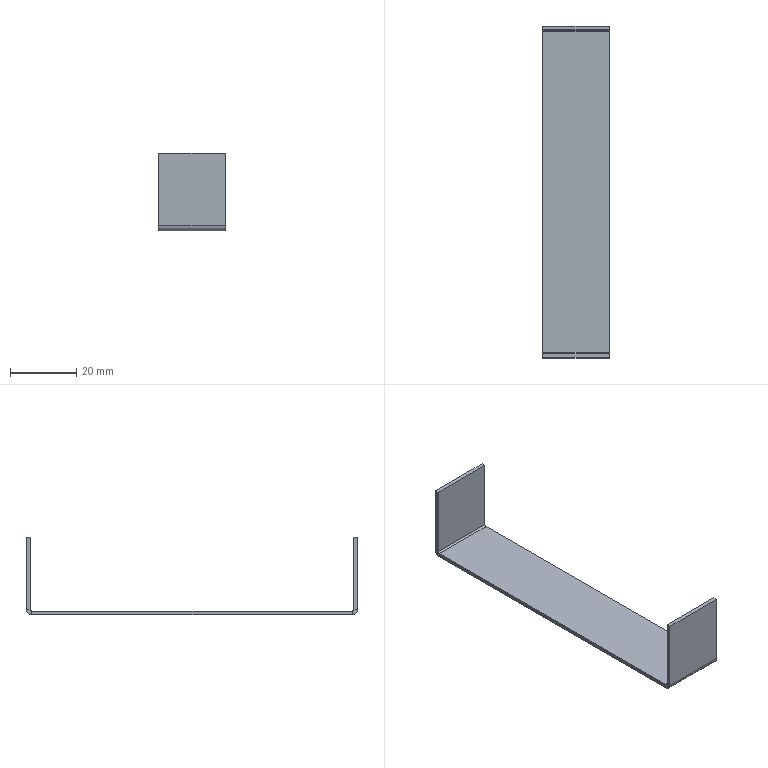Component | SolidWorks | AirFurnaceElectricalCabinet-DoorPanelAssembly-1_AirFurnaceElectricalCabinet-WiringBoard-2 | 1 solid | 22 faces | box 20 x 100 x 23.5 mm | volume 3448 mm3 | plane 18 | cylinder 4 | commonest cylinder face diameters 3.4 x2 1 x2
STEP:
#1=COLOUR_RGB('',0.7922,0.8196,0.9333);
#2=FILL_AREA_STYLE_COLOUR('',#1);
#3=FILL_AREA_STYLE('',(#2));
#4=SURFACE_STYLE_FILL_AREA(#3);
#5=SURFACE_SIDE_STYLE('',(#4));
#6=SURFACE_STYLE_USAGE(.BOTH.,#5);
#7=PRESENTATION_STYLE_ASSIGNMENT((#6));
#8=CARTESIAN_POINT('',(-18.504,43.728,9.055));
#9=VERTEX_POINT('',#8);
#10=CARTESIAN_POINT('',(-18.504,43.728,9.102));
#11=VERTEX_POINT('',#10);
#12=CARTESIAN_POINT('',(-18.504,43.728,9.055));
#13=DIRECTION('',(-0.,-0.,1.));
#14=VECTOR('',#13,39.37);
#15=LINE('',#12,#14);
#16=EDGE_CURVE('',#9,#11,#15,.T.);
#17=ORIENTED_EDGE('',*,*,#16,.F.);
#18=CARTESIAN_POINT('',(-18.504,43.661,9.122));
#19=VERTEX_POINT('',#18);
#20=CARTESIAN_POINT('',(-18.504,43.728,9.122));
#21=DIRECTION('',(1.,-0.,0.));
#22=DIRECTION('',(0.,1.,0.));
#23=AXIS2_PLACEMENT_3D('',#20,#21,#22);
#24=CIRCLE('',#23,0.06693);
#25=EDGE_CURVE('',#19,#9,#24,.T.);
#26=ORIENTED_EDGE('',*,*,#25,.F.);
#27=CARTESIAN_POINT('',(-18.504,43.709,9.122));
#28=VERTEX_POINT('',#27);
#29=CARTESIAN_POINT('',(-18.504,43.709,9.122));
#30=DIRECTION('',(-0.,-1.,-0.));
#31=VECTOR('',#30,39.37);
#32=LINE('',#29,#31);
#33=EDGE_CURVE('',#28,#19,#32,.T.);
#34=ORIENTED_EDGE('',*,*,#33,.F.);
#35=CARTESIAN_POINT('',(-18.504,43.728,9.122));
#36=DIRECTION('',(1.,-0.,0.));
#37=DIRECTION('',(0.,1.,0.));
#38=AXIS2_PLACEMENT_3D('',#35,#36,#37);
#39=CIRCLE('',#38,0.01969);
#40=EDGE_CURVE('',#28,#11,#39,.T.);
#41=ORIENTED_EDGE('',*,*,#40,.T.);
#42=EDGE_LOOP('',(#17,#26,#34,#41));
#43=FACE_OUTER_BOUND('',#42,.T.);
#44=CARTESIAN_POINT('',(-18.504,43.728,9.055));
#45=DIRECTION('',(-1.,0.,-0.));
#46=DIRECTION('',(0.,1.,0.));
#47=AXIS2_PLACEMENT_3D('',#44,#45,#46);
#48=PLANE('',#47);
#49=ADVANCED_FACE('',(#43),#48,.T.);
#50=CARTESIAN_POINT('',(-18.504,47.531,9.055));
#51=VERTEX_POINT('',#50);
#52=CARTESIAN_POINT('',(-18.504,43.661,9.055));
#53=DIRECTION('',(0.,1.,0.));
#54=VECTOR('',#53,39.37);
#55=LINE('',#52,#54);
#56=EDGE_CURVE('',#9,#51,#55,.T.);
#57=ORIENTED_EDGE('',*,*,#56,.F.);
#58=ORIENTED_EDGE('',*,*,#16,.T.);
#59=CARTESIAN_POINT('',(-18.504,47.531,9.102));
#60=VERTEX_POINT('',#59);
#61=CARTESIAN_POINT('',(-18.504,43.661,9.102));
#62=DIRECTION('',(0.,1.,0.));
#63=VECTOR('',#62,39.37);
#64=LINE('',#61,#63);
#65=EDGE_CURVE('',#11,#60,#64,.T.);
#66=ORIENTED_EDGE('',*,*,#65,.T.);
#67=CARTESIAN_POINT('',(-18.504,47.531,9.102));
#68=DIRECTION('',(0.,0.,-1.));
#69=VECTOR('',#68,39.37);
#70=LINE('',#67,#69);
#71=EDGE_CURVE('',#60,#51,#70,.T.);
#72=ORIENTED_EDGE('',*,*,#71,.T.);
#73=EDGE_LOOP('',(#57,#58,#66,#72));
#74=FACE_OUTER_BOUND('',#73,.T.);
#75=CARTESIAN_POINT('',(-18.504,43.709,9.122));
#76=DIRECTION('',(-1.,0.,-0.));
#77=DIRECTION('',(0.,1.,0.));
#78=AXIS2_PLACEMENT_3D('',#75,#76,#77);
#79=PLANE('',#78);
#80=ADVANCED_FACE('',(#74),#79,.T.);
#81=CARTESIAN_POINT('',(-17.717,43.661,9.122));
#82=VERTEX_POINT('',#81);
#83=CARTESIAN_POINT('',(-17.717,43.709,9.122));
#84=VERTEX_POINT('',#83);
#85=CARTESIAN_POINT('',(-17.717,43.661,9.122));
#86=DIRECTION('',(0.,1.,0.));
#87=VECTOR('',#86,39.37);
#88=LINE('',#85,#87);
#89=EDGE_CURVE('',#82,#84,#88,.T.);
#90=ORIENTED_EDGE('',*,*,#89,.F.);
#91=CARTESIAN_POINT('',(-17.717,43.728,9.055));
#92=VERTEX_POINT('',#91);
#93=CARTESIAN_POINT('',(-17.717,43.728,9.122));
#94=DIRECTION('',(1.,-0.,0.));
#95=DIRECTION('',(0.,1.,0.));
#96=AXIS2_PLACEMENT_3D('',#93,#94,#95);
#97=CIRCLE('',#96,0.06693);
#98=EDGE_CURVE('',#82,#92,#97,.T.);
#99=ORIENTED_EDGE('',*,*,#98,.T.);
#100=CARTESIAN_POINT('',(-17.717,43.728,9.102));
#101=VERTEX_POINT('',#100);
#102=CARTESIAN_POINT('',(-17.717,43.728,9.102));
#103=DIRECTION('',(0.,0.,-1.));
#104=VECTOR('',#103,39.37);
#105=LINE('',#102,#104);
#106=EDGE_CURVE('',#101,#92,#105,.T.);
#107=ORIENTED_EDGE('',*,*,#106,.F.);
#108=CARTESIAN_POINT('',(-17.717,43.728,9.122));
#109=DIRECTION('',(1.,-0.,0.));
#110=DIRECTION('',(0.,1.,0.));
#111=AXIS2_PLACEMENT_3D('',#108,#109,#110);
#112=CIRCLE('',#111,0.01969);
#113=EDGE_CURVE('',#84,#101,#112,.T.);
#114=ORIENTED_EDGE('',*,*,#113,.F.);
#115=EDGE_LOOP('',(#90,#99,#107,#114));
#116=FACE_OUTER_BOUND('',#115,.T.);
#117=CARTESIAN_POINT('',(-17.717,43.661,9.122));
#118=DIRECTION('',(1.,-0.,0.));
#119=DIRECTION('',(-0.,-1.,-0.));
#120=AXIS2_PLACEMENT_3D('',#117,#118,#119);
#121=PLANE('',#120);
#122=ADVANCED_FACE('',(#116),#121,.T.);
#123=CARTESIAN_POINT('',(-17.717,43.661,9.98));
#124=VERTEX_POINT('',#123);
#125=CARTESIAN_POINT('',(-17.717,43.661,9.98));
#126=DIRECTION('',(0.,0.,-1.));
#127=VECTOR('',#126,39.37);
#128=LINE('',#125,#127);
#129=EDGE_CURVE('',#124,#82,#128,.T.);
#130=ORIENTED_EDGE('',*,*,#129,.T.);
#131=ORIENTED_EDGE('',*,*,#89,.T.);
#132=CARTESIAN_POINT('',(-17.717,43.709,9.98));
#133=VERTEX_POINT('',#132);
#134=CARTESIAN_POINT('',(-17.717,43.709,9.98));
#135=DIRECTION('',(0.,0.,-1.));
#136=VECTOR('',#135,39.37);
#137=LINE('',#134,#136);
#138=EDGE_CURVE('',#133,#84,#137,.T.);
#139=ORIENTED_EDGE('',*,*,#138,.F.);
#140=CARTESIAN_POINT('',(-17.717,43.709,9.98));
#141=DIRECTION('',(-0.,-1.,-0.));
#142=VECTOR('',#141,39.37);
#143=LINE('',#140,#142);
#144=EDGE_CURVE('',#133,#124,#143,.T.);
#145=ORIENTED_EDGE('',*,*,#144,.T.);
#146=EDGE_LOOP('',(#130,#131,#139,#145));
#147=FACE_OUTER_BOUND('',#146,.T.);
#148=CARTESIAN_POINT('',(-17.717,43.728,9.102));
#149=DIRECTION('',(1.,-0.,0.));
#150=DIRECTION('',(-0.,-1.,-0.));
#151=AXIS2_PLACEMENT_3D('',#148,#149,#150);
#152=PLANE('',#151);
#153=ADVANCED_FACE('',(#147),#152,.T.);
#154=CARTESIAN_POINT('',(-18.504,47.598,9.122));
#155=VERTEX_POINT('',#154);
#156=CARTESIAN_POINT('',(-18.504,47.551,9.122));
#157=VERTEX_POINT('',#156);
#158=CARTESIAN_POINT('',(-18.504,47.598,9.122));
#159=DIRECTION('',(-0.,-1.,-0.));
#160=VECTOR('',#159,39.37);
#161=LINE('',#158,#160);
#162=EDGE_CURVE('',#155,#157,#161,.T.);
#163=ORIENTED_EDGE('',*,*,#162,.F.);
#164=CARTESIAN_POINT('',(-18.504,47.531,9.122));
#165=DIRECTION('',(1.,-0.,0.));
#166=DIRECTION('',(0.,1.,0.));
#167=AXIS2_PLACEMENT_3D('',#164,#165,#166);
#168=CIRCLE('',#167,0.06693);
#169=EDGE_CURVE('',#51,#155,#168,.T.);
#170=ORIENTED_EDGE('',*,*,#169,.F.);
#171=ORIENTED_EDGE('',*,*,#71,.F.);
#172=CARTESIAN_POINT('',(-18.504,47.531,9.122));
#173=DIRECTION('',(1.,-0.,0.));
#174=DIRECTION('',(0.,1.,0.));
#175=AXIS2_PLACEMENT_3D('',#172,#173,#174);
#176=CIRCLE('',#175,0.01969);
#177=EDGE_CURVE('',#60,#157,#176,.T.);
#178=ORIENTED_EDGE('',*,*,#177,.T.);
#179=EDGE_LOOP('',(#163,#170,#171,#178));
#180=FACE_OUTER_BOUND('',#179,.T.);
#181=CARTESIAN_POINT('',(-18.504,47.598,9.122));
#182=DIRECTION('',(-1.,0.,-0.));
#183=DIRECTION('',(0.,1.,0.));
#184=AXIS2_PLACEMENT_3D('',#181,#182,#183);
#185=PLANE('',#184);
#186=ADVANCED_FACE('',(#180),#185,.T.);
#187=CARTESIAN_POINT('',(-18.504,47.598,9.98));
#188=VERTEX_POINT('',#187);
#189=CARTESIAN_POINT('',(-18.504,47.598,9.055));
#190=DIRECTION('',(-0.,-0.,1.));
#191=VECTOR('',#190,39.37);
#192=LINE('',#189,#191);
#193=EDGE_CURVE('',#155,#188,#192,.T.);
#194=ORIENTED_EDGE('',*,*,#193,.F.);
#195=ORIENTED_EDGE('',*,*,#162,.T.);
#196=CARTESIAN_POINT('',(-18.504,47.551,9.98));
#197=VERTEX_POINT('',#196);
#198=CARTESIAN_POINT('',(-18.504,47.551,9.055));
#199=DIRECTION('',(-0.,-0.,1.));
#200=VECTOR('',#199,39.37);
#201=LINE('',#198,#200);
#202=EDGE_CURVE('',#157,#197,#201,.T.);
#203=ORIENTED_EDGE('',*,*,#202,.T.);
#204=CARTESIAN_POINT('',(-18.504,47.598,9.98));
#205=DIRECTION('',(-0.,-1.,-0.));
#206=VECTOR('',#205,39.37);
#207=LINE('',#204,#206);
#208=EDGE_CURVE('',#188,#197,#207,.T.);
#209=ORIENTED_EDGE('',*,*,#208,.F.);
#210=EDGE_LOOP('',(#194,#195,#203,#209));
#211=FACE_OUTER_BOUND('',#210,.T.);
#212=CARTESIAN_POINT('',(-18.504,47.531,9.102));
#213=DIRECTION('',(-1.,0.,-0.));
#214=DIRECTION('',(0.,1.,0.));
#215=AXIS2_PLACEMENT_3D('',#212,#213,#214);
#216=PLANE('',#215);
#217=ADVANCED_FACE('',(#211),#216,.T.);
#218=CARTESIAN_POINT('',(-17.717,47.531,9.055));
#219=VERTEX_POINT('',#218);
#220=CARTESIAN_POINT('',(-17.717,47.531,9.102));
#221=VERTEX_POINT('',#220);
#222=CARTESIAN_POINT('',(-17.717,47.531,9.055));
#223=DIRECTION('',(-0.,-0.,1.));
#224=VECTOR('',#223,39.37);
#225=LINE('',#222,#224);
#226=EDGE_CURVE('',#219,#221,#225,.T.);
#227=ORIENTED_EDGE('',*,*,#226,.F.);
#228=CARTESIAN_POINT('',(-17.717,47.598,9.122));
#229=VERTEX_POINT('',#228);
#230=CARTESIAN_POINT('',(-17.717,47.531,9.122));
#231=DIRECTION('',(1.,-0.,0.));
#232=DIRECTION('',(0.,1.,0.));
#233=AXIS2_PLACEMENT_3D('',#230,#231,#232);
#234=CIRCLE('',#233,0.06693);
#235=EDGE_CURVE('',#219,#229,#234,.T.);
#236=ORIENTED_EDGE('',*,*,#235,.T.);
#237=CARTESIAN_POINT('',(-17.717,47.551,9.122));
#238=VERTEX_POINT('',#237);
#239=CARTESIAN_POINT('',(-17.717,47.551,9.122));
#240=DIRECTION('',(0.,1.,0.));
#241=VECTOR('',#240,39.37);
#242=LINE('',#239,#241);
#243=EDGE_CURVE('',#238,#229,#242,.T.);
#244=ORIENTED_EDGE('',*,*,#243,.F.);
#245=CARTESIAN_POINT('',(-17.717,47.531,9.122));
#246=DIRECTION('',(1.,-0.,0.));
#247=DIRECTION('',(0.,1.,0.));
#248=AXIS2_PLACEMENT_3D('',#245,#246,#247);
#249=CIRCLE('',#248,0.01969);
#250=EDGE_CURVE('',#221,#238,#249,.T.);
#251=ORIENTED_EDGE('',*,*,#250,.F.);
#252=EDGE_LOOP('',(#227,#236,#244,#251));
#253=FACE_OUTER_BOUND('',#252,.T.);
#254=CARTESIAN_POINT('',(-17.717,47.531,9.055));
#255=DIRECTION('',(1.,-0.,0.));
#256=DIRECTION('',(-0.,-1.,-0.));
#257=AXIS2_PLACEMENT_3D('',#254,#255,#256);
#258=PLANE('',#257);
#259=ADVANCED_FACE('',(#253),#258,.T.);
#260=CARTESIAN_POINT('',(-17.717,43.661,9.055));
#261=DIRECTION('',(0.,1.,0.));
#262=VECTOR('',#261,39.37);
#263=LINE('',#260,#262);
#264=EDGE_CURVE('',#92,#219,#263,.T.);
#265=ORIENTED_EDGE('',*,*,#264,.T.);
#266=ORIENTED_EDGE('',*,*,#226,.T.);
#267=CARTESIAN_POINT('',(-17.717,43.661,9.102));
#268=DIRECTION('',(0.,1.,0.));
#269=VECTOR('',#268,39.37);
#270=LINE('',#267,#269);
#271=EDGE_CURVE('',#101,#221,#270,.T.);
#272=ORIENTED_EDGE('',*,*,#271,.F.);
#273=ORIENTED_EDGE('',*,*,#106,.T.);
#274=EDGE_LOOP('',(#265,#266,#272,#273));
#275=FACE_OUTER_BOUND('',#274,.T.);
#276=CARTESIAN_POINT('',(-17.717,47.551,9.122));
#277=DIRECTION('',(1.,-0.,0.));
#278=DIRECTION('',(-0.,-1.,-0.));
#279=AXIS2_PLACEMENT_3D('',#276,#277,#278);
#280=PLANE('',#279);
#281=ADVANCED_FACE('',(#275),#280,.T.);
#282=CARTESIAN_POINT('',(-17.717,47.551,9.98));
#283=VERTEX_POINT('',#282);
#284=CARTESIAN_POINT('',(-17.717,47.551,9.055));
#285=DIRECTION('',(-0.,-0.,1.));
#286=VECTOR('',#285,39.37);
#287=LINE('',#284,#286);
#288=EDGE_CURVE('',#238,#283,#287,.T.);
#289=ORIENTED_EDGE('',*,*,#288,.T.);
#290=CARTESIAN_POINT('',(-18.504,47.551,9.98));
#291=DIRECTION('',(1.,-0.,0.));
#292=VECTOR('',#291,39.37);
#293=LINE('',#290,#292);
#294=EDGE_CURVE('',#197,#283,#293,.T.);
#295=ORIENTED_EDGE('',*,*,#294,.F.);
#296=ORIENTED_EDGE('',*,*,#202,.F.);
#297=CARTESIAN_POINT('',(-18.504,47.551,9.122));
#298=DIRECTION('',(1.,-0.,0.));
#299=VECTOR('',#298,39.37);
#300=LINE('',#297,#299);
#301=EDGE_CURVE('',#157,#238,#300,.T.);
#302=ORIENTED_EDGE('',*,*,#301,.T.);
#303=EDGE_LOOP('',(#289,#295,#296,#302));
#304=FACE_OUTER_BOUND('',#303,.T.);
#305=CARTESIAN_POINT('',(-18.504,47.551,9.055));
#306=DIRECTION('',(0.,1.,0.));
#307=DIRECTION('',(0.,0.,-1.));
#308=AXIS2_PLACEMENT_3D('',#305,#306,#307);
#309=PLANE('',#308);
#310=ADVANCED_FACE('',(#304),#309,.F.);
#311=CARTESIAN_POINT('',(-17.717,47.598,9.98));
#312=VERTEX_POINT('',#311);
#313=CARTESIAN_POINT('',(-17.717,47.598,9.98));
#314=DIRECTION('',(-0.,-1.,-0.));
#315=VECTOR('',#314,39.37);
#316=LINE('',#313,#315);
#317=EDGE_CURVE('',#312,#283,#316,.T.);
#318=ORIENTED_EDGE('',*,*,#317,.F.);
#319=CARTESIAN_POINT('',(-18.504,47.598,9.98));
#320=DIRECTION('',(1.,-0.,0.));
#321=VECTOR('',#320,39.37);
#322=LINE('',#319,#321);
#323=EDGE_CURVE('',#188,#312,#322,.T.);
#324=ORIENTED_EDGE('',*,*,#323,.F.);
#325=ORIENTED_EDGE('',*,*,#208,.T.);
#326=ORIENTED_EDGE('',*,*,#294,.T.);
#327=EDGE_LOOP('',(#318,#324,#325,#326));
#328=FACE_OUTER_BOUND('',#327,.T.);
#329=CARTESIAN_POINT('',(-18.504,47.598,9.98));
#330=DIRECTION('',(-0.,-0.,1.));
#331=DIRECTION('',(0.,1.,0.));
#332=AXIS2_PLACEMENT_3D('',#329,#330,#331);
#333=PLANE('',#332);
#334=ADVANCED_FACE('',(#328),#333,.T.);
#335=CARTESIAN_POINT('',(-17.717,47.598,9.055));
#336=DIRECTION('',(-0.,-0.,1.));
#337=VECTOR('',#336,39.37);
#338=LINE('',#335,#337);
#339=EDGE_CURVE('',#229,#312,#338,.T.);
#340=ORIENTED_EDGE('',*,*,#339,.F.);
#341=CARTESIAN_POINT('',(-18.504,47.598,9.122));
#342=DIRECTION('',(1.,-0.,0.));
#343=VECTOR('',#342,39.37);
#344=LINE('',#341,#343);
#345=EDGE_CURVE('',#155,#229,#344,.T.);
#346=ORIENTED_EDGE('',*,*,#345,.F.);
#347=ORIENTED_EDGE('',*,*,#193,.T.);
#348=ORIENTED_EDGE('',*,*,#323,.T.);
#349=EDGE_LOOP('',(#340,#346,#347,#348));
#350=FACE_OUTER_BOUND('',#349,.T.);
#351=CARTESIAN_POINT('',(-18.504,47.598,9.055));
#352=DIRECTION('',(0.,1.,0.));
#353=DIRECTION('',(0.,0.,-1.));
#354=AXIS2_PLACEMENT_3D('',#351,#352,#353);
#355=PLANE('',#354);
#356=ADVANCED_FACE('',(#350),#355,.T.);
#357=ORIENTED_EDGE('',*,*,#235,.F.);
#358=CARTESIAN_POINT('',(-18.504,47.531,9.055));
#359=DIRECTION('',(1.,-0.,0.));
#360=VECTOR('',#359,39.37);
#361=LINE('',#358,#360);
#362=EDGE_CURVE('',#51,#219,#361,.T.);
#363=ORIENTED_EDGE('',*,*,#362,.F.);
#364=ORIENTED_EDGE('',*,*,#169,.T.);
#365=ORIENTED_EDGE('',*,*,#345,.T.);
#366=EDGE_LOOP('',(#357,#363,#364,#365));
#367=FACE_OUTER_BOUND('',#366,.T.);
#368=CARTESIAN_POINT('',(-18.504,47.531,9.122));
#369=DIRECTION('',(1.,-0.,0.));
#370=DIRECTION('',(0.,-1.,0.));
#371=AXIS2_PLACEMENT_3D('',#368,#369,#370);
#372=CYLINDRICAL_SURFACE('',#371,0.06693);
#373=ADVANCED_FACE('',(#367),#372,.T.);
#374=ORIENTED_EDGE('',*,*,#264,.F.);
#375=CARTESIAN_POINT('',(-18.504,43.728,9.055));
#376=DIRECTION('',(1.,-0.,0.));
#377=VECTOR('',#376,39.37);
#378=LINE('',#375,#377);
#379=EDGE_CURVE('',#9,#92,#378,.T.);
#380=ORIENTED_EDGE('',*,*,#379,.F.);
#381=ORIENTED_EDGE('',*,*,#56,.T.);
#382=ORIENTED_EDGE('',*,*,#362,.T.);
#383=EDGE_LOOP('',(#374,#380,#381,#382));
#384=FACE_OUTER_BOUND('',#383,.T.);
#385=CARTESIAN_POINT('',(-18.504,43.661,9.055));
#386=DIRECTION('',(0.,0.,-1.));
#387=DIRECTION('',(-0.,-1.,-0.));
#388=AXIS2_PLACEMENT_3D('',#385,#386,#387);
#389=PLANE('',#388);
#390=ADVANCED_FACE('',(#384),#389,.T.);
#391=ORIENTED_EDGE('',*,*,#98,.F.);
#392=CARTESIAN_POINT('',(-18.504,43.661,9.122));
#393=DIRECTION('',(1.,-0.,0.));
#394=VECTOR('',#393,39.37);
#395=LINE('',#392,#394);
#396=EDGE_CURVE('',#19,#82,#395,.T.);
#397=ORIENTED_EDGE('',*,*,#396,.F.);
#398=ORIENTED_EDGE('',*,*,#25,.T.);
#399=ORIENTED_EDGE('',*,*,#379,.T.);
#400=EDGE_LOOP('',(#391,#397,#398,#399));
#401=FACE_OUTER_BOUND('',#400,.T.);
#402=CARTESIAN_POINT('',(-18.504,43.728,9.122));
#403=DIRECTION('',(1.,-0.,0.));
#404=DIRECTION('',(0.,-1.,0.));
#405=AXIS2_PLACEMENT_3D('',#402,#403,#404);
#406=CYLINDRICAL_SURFACE('',#405,0.06693);
#407=ADVANCED_FACE('',(#401),#406,.T.);
#408=ORIENTED_EDGE('',*,*,#129,.F.);
#409=CARTESIAN_POINT('',(-18.504,43.661,9.98));
#410=VERTEX_POINT('',#409);
#411=CARTESIAN_POINT('',(-18.504,43.661,9.98));
#412=DIRECTION('',(1.,-0.,0.));
#413=VECTOR('',#412,39.37);
#414=LINE('',#411,#413);
#415=EDGE_CURVE('',#410,#124,#414,.T.);
#416=ORIENTED_EDGE('',*,*,#415,.F.);
#417=CARTESIAN_POINT('',(-18.504,43.661,9.98));
#418=DIRECTION('',(0.,0.,-1.));
#419=VECTOR('',#418,39.37);
#420=LINE('',#417,#419);
#421=EDGE_CURVE('',#410,#19,#420,.T.);
#422=ORIENTED_EDGE('',*,*,#421,.T.);
#423=ORIENTED_EDGE('',*,*,#396,.T.);
#424=EDGE_LOOP('',(#408,#416,#422,#423));
#425=FACE_OUTER_BOUND('',#424,.T.);
#426=CARTESIAN_POINT('',(-18.504,43.661,9.98));
#427=DIRECTION('',(0.,-1.,-0.));
#428=DIRECTION('',(-1.,0.,-0.));
#429=AXIS2_PLACEMENT_3D('',#426,#427,#428);
#430=PLANE('',#429);
#431=ADVANCED_FACE('',(#425),#430,.T.);
#432=ORIENTED_EDGE('',*,*,#144,.F.);
#433=CARTESIAN_POINT('',(-18.504,43.709,9.98));
#434=VERTEX_POINT('',#433);
#435=CARTESIAN_POINT('',(-18.504,43.709,9.98));
#436=DIRECTION('',(1.,-0.,0.));
#437=VECTOR('',#436,39.37);
#438=LINE('',#435,#437);
#439=EDGE_CURVE('',#434,#133,#438,.T.);
#440=ORIENTED_EDGE('',*,*,#439,.F.);
#441=CARTESIAN_POINT('',(-18.504,43.709,9.98));
#442=DIRECTION('',(-0.,-1.,-0.));
#443=VECTOR('',#442,39.37);
#444=LINE('',#441,#443);
#445=EDGE_CURVE('',#434,#410,#444,.T.);
#446=ORIENTED_EDGE('',*,*,#445,.T.);
#447=ORIENTED_EDGE('',*,*,#415,.T.);
#448=EDGE_LOOP('',(#432,#440,#446,#447));
#449=FACE_OUTER_BOUND('',#448,.T.);
#450=CARTESIAN_POINT('',(-18.504,43.709,9.98));
#451=DIRECTION('',(-0.,-0.,1.));
#452=DIRECTION('',(1.,-0.,0.));
#453=AXIS2_PLACEMENT_3D('',#450,#451,#452);
#454=PLANE('',#453);
#455=ADVANCED_FACE('',(#449),#454,.T.);
#456=ORIENTED_EDGE('',*,*,#138,.T.);
#457=CARTESIAN_POINT('',(-18.504,43.709,9.122));
#458=DIRECTION('',(1.,-0.,0.));
#459=VECTOR('',#458,39.37);
#460=LINE('',#457,#459);
#461=EDGE_CURVE('',#28,#84,#460,.T.);
#462=ORIENTED_EDGE('',*,*,#461,.F.);
#463=CARTESIAN_POINT('',(-18.504,43.709,9.98));
#464=DIRECTION('',(0.,0.,-1.));
#465=VECTOR('',#464,39.37);
#466=LINE('',#463,#465);
#467=EDGE_CURVE('',#434,#28,#466,.T.);
#468=ORIENTED_EDGE('',*,*,#467,.F.);
#469=ORIENTED_EDGE('',*,*,#439,.T.);
#470=EDGE_LOOP('',(#456,#462,#468,#469));
#471=FACE_OUTER_BOUND('',#470,.T.);
#472=CARTESIAN_POINT('',(-18.504,43.709,9.98));
#473=DIRECTION('',(0.,-1.,-0.));
#474=DIRECTION('',(-1.,0.,-0.));
#475=AXIS2_PLACEMENT_3D('',#472,#473,#474);
#476=PLANE('',#475);
#477=ADVANCED_FACE('',(#471),#476,.F.);
#478=ORIENTED_EDGE('',*,*,#113,.T.);
#479=CARTESIAN_POINT('',(-18.504,43.728,9.102));
#480=DIRECTION('',(1.,-0.,0.));
#481=VECTOR('',#480,39.37);
#482=LINE('',#479,#481);
#483=EDGE_CURVE('',#11,#101,#482,.T.);
#484=ORIENTED_EDGE('',*,*,#483,.F.);
#485=ORIENTED_EDGE('',*,*,#40,.F.);
#486=ORIENTED_EDGE('',*,*,#461,.T.);
#487=EDGE_LOOP('',(#478,#484,#485,#486));
#488=FACE_OUTER_BOUND('',#487,.T.);
#489=CARTESIAN_POINT('',(-18.504,43.728,9.122));
#490=DIRECTION('',(1.,-0.,0.));
#491=DIRECTION('',(0.,-1.,0.));
#492=AXIS2_PLACEMENT_3D('',#489,#490,#491);
#493=CYLINDRICAL_SURFACE('',#492,0.01969);
#494=ADVANCED_FACE('',(#488),#493,.F.);
#495=ORIENTED_EDGE('',*,*,#271,.T.);
#496=CARTESIAN_POINT('',(-18.504,47.531,9.102));
#497=DIRECTION('',(1.,-0.,0.));
#498=VECTOR('',#497,39.37);
#499=LINE('',#496,#498);
#500=EDGE_CURVE('',#60,#221,#499,.T.);
#501=ORIENTED_EDGE('',*,*,#500,.F.);
#502=ORIENTED_EDGE('',*,*,#65,.F.);
#503=ORIENTED_EDGE('',*,*,#483,.T.);
#504=EDGE_LOOP('',(#495,#501,#502,#503));
#505=FACE_OUTER_BOUND('',#504,.T.);
#506=CARTESIAN_POINT('',(-18.504,43.661,9.102));
#507=DIRECTION('',(0.,0.,-1.));
#508=DIRECTION('',(-0.,-1.,-0.));
#509=AXIS2_PLACEMENT_3D('',#506,#507,#508);
#510=PLANE('',#509);
#511=ADVANCED_FACE('',(#505),#510,.F.);
#512=ORIENTED_EDGE('',*,*,#250,.T.);
#513=ORIENTED_EDGE('',*,*,#301,.F.);
#514=ORIENTED_EDGE('',*,*,#177,.F.);
#515=ORIENTED_EDGE('',*,*,#500,.T.);
#516=EDGE_LOOP('',(#512,#513,#514,#515));
#517=FACE_OUTER_BOUND('',#516,.T.);
#518=CARTESIAN_POINT('',(-18.504,47.531,9.122));
#519=DIRECTION('',(1.,-0.,0.));
#520=DIRECTION('',(0.,-1.,0.));
#521=AXIS2_PLACEMENT_3D('',#518,#519,#520);
#522=CYLINDRICAL_SURFACE('',#521,0.01969);
#523=ADVANCED_FACE('',(#517),#522,.F.);
#524=ORIENTED_EDGE('',*,*,#467,.T.);
#525=ORIENTED_EDGE('',*,*,#33,.T.);
#526=ORIENTED_EDGE('',*,*,#421,.F.);
#527=ORIENTED_EDGE('',*,*,#445,.F.);
#528=EDGE_LOOP('',(#524,#525,#526,#527));
#529=FACE_OUTER_BOUND('',#528,.T.);
#530=CARTESIAN_POINT('',(-18.504,47.531,9.122));
#531=DIRECTION('',(-1.,0.,-0.));
#532=DIRECTION('',(0.,1.,0.));
#533=AXIS2_PLACEMENT_3D('',#530,#531,#532);
#534=PLANE('',#533);
#535=ADVANCED_FACE('',(#529),#534,.T.);
#536=ORIENTED_EDGE('',*,*,#288,.F.);
#537=ORIENTED_EDGE('',*,*,#243,.T.);
#538=ORIENTED_EDGE('',*,*,#339,.T.);
#539=ORIENTED_EDGE('',*,*,#317,.T.);
#540=EDGE_LOOP('',(#536,#537,#538,#539));
#541=FACE_OUTER_BOUND('',#540,.T.);
#542=CARTESIAN_POINT('',(-17.717,47.531,9.122));
#543=DIRECTION('',(-1.,0.,-0.));
#544=DIRECTION('',(0.,1.,0.));
#545=AXIS2_PLACEMENT_3D('',#542,#543,#544);
#546=PLANE('',#545);
#547=ADVANCED_FACE('',(#541),#546,.F.);
#548=CLOSED_SHELL('',(#49,#80,#122,#153,#186,#217,#259,#281,#310,#334,#356,#373,#390,#407,#431,#455,#477,#494,#511,#523,#535,#547));
#549=MANIFOLD_SOLID_BREP('',#548);
#550=STYLED_ITEM('',(#7),#549);
#551=PRESENTATION_LAYER_ASSIGNMENT('','',(#550));
#552=(LENGTH_UNIT()NAMED_UNIT(*)SI_UNIT($,.METRE.));
#553=LENGTH_MEASURE_WITH_UNIT(LENGTH_MEASURE(0.0254),#552);
#554=DIMENSIONAL_EXPONENTS(1.,0.,0.,0.,0.,0.,0.);
#555=(CONVERSION_BASED_UNIT('',#553)LENGTH_UNIT()NAMED_UNIT(#554));
#556=UNCERTAINTY_MEASURE_WITH_UNIT(LENGTH_MEASURE(0.00001),#555,'','');
#557=(NAMED_UNIT(*)PLANE_ANGLE_UNIT()SI_UNIT($,.RADIAN.));
#558=(NAMED_UNIT(*)SI_UNIT($,.STERADIAN.)SOLID_ANGLE_UNIT());
#559=(GEOMETRIC_REPRESENTATION_CONTEXT(3)GLOBAL_UNCERTAINTY_ASSIGNED_CONTEXT((#556))GLOBAL_UNIT_ASSIGNED_CONTEXT((#555,#557,#558))REPRESENTATION_CONTEXT('',''));
#560=MECHANICAL_DESIGN_GEOMETRIC_PRESENTATION_REPRESENTATION('',(#550),#559);
#561=CARTESIAN_POINT('',(0.,0.,0.));
#562=DIRECTION('',(0.,0.,1.));
#563=DIRECTION('',(1.,0.,0.));
#564=AXIS2_PLACEMENT_3D('',#561,#562,#563);
#565=(LENGTH_UNIT()NAMED_UNIT(*)SI_UNIT($,.METRE.));
#566=LENGTH_MEASURE_WITH_UNIT(LENGTH_MEASURE(0.0254),#565);
#567=DIMENSIONAL_EXPONENTS(1.,0.,0.,0.,0.,0.,0.);
#568=(CONVERSION_BASED_UNIT('',#566)LENGTH_UNIT()NAMED_UNIT(#567));
#569=UNCERTAINTY_MEASURE_WITH_UNIT(LENGTH_MEASURE(0.00001),#568,'','');
#570=(NAMED_UNIT(*)PLANE_ANGLE_UNIT()SI_UNIT($,.RADIAN.));
#571=(NAMED_UNIT(*)SI_UNIT($,.STERADIAN.)SOLID_ANGLE_UNIT());
#572=(GEOMETRIC_REPRESENTATION_CONTEXT(3)GLOBAL_UNCERTAINTY_ASSIGNED_CONTEXT((#569))GLOBAL_UNIT_ASSIGNED_CONTEXT((#568,#570,#571))REPRESENTATION_CONTEXT('',''));
#573=ADVANCED_BREP_SHAPE_REPRESENTATION('',(#549,#564),#572);